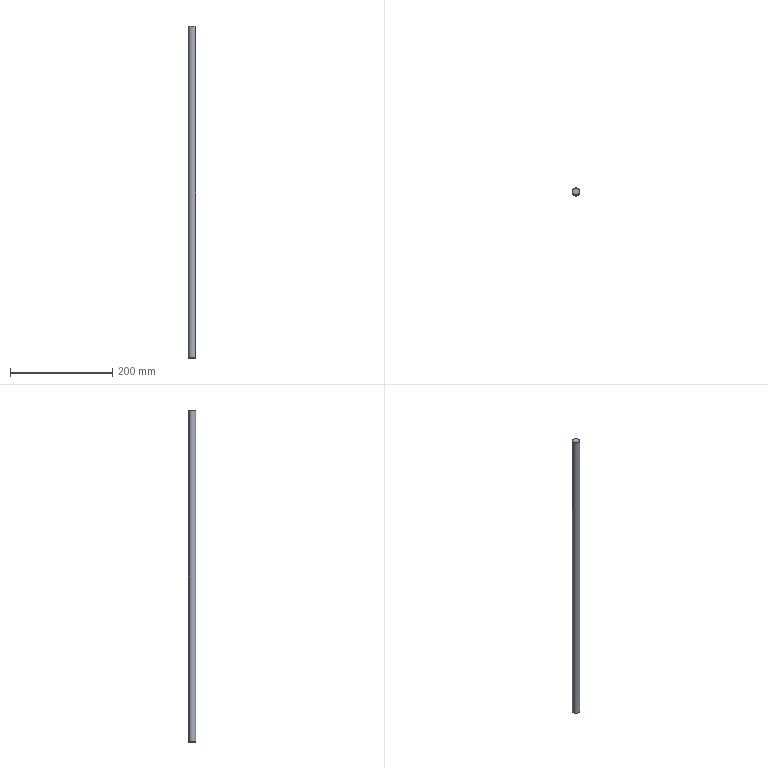Component | SolidWorks | KSD171005A-01-01-18-1 | 1 solid | 8 faces | box 15 x 15 x 650 mm | volume 114819 mm3 | cone 4 | cylinder 2 | plane 2 | commonest cylinder face diameters 15 x2
build123d program:
from build123d import *

# Parameters (mm, degrees)
SKETCH1_R           = 7.5
BOSS_EXTRUDE1_DEPTH = 650
CHAMFER1_SIZE       = 1


with BuildPart() as part:
    # Sketch1 → Boss-Extrude1 (new body)
    with BuildSketch(Plane.XY):
        Circle(SKETCH1_R)
    extrude(amount=BOSS_EXTRUDE1_DEPTH)

    # Chamfer1
    chamfer1_edges = [part.edges().sort_by_distance(p)[0] for p in [
        (-7.5, 0, 0),
        (-7.5, 0, 650),
    ]]
    chamfer(chamfer1_edges, length=CHAMFER1_SIZE)


solid = part.part

# Placed as in the assembly
solid = solid.moved(Location((-7.111, 15.73, 328), (0, 0, 0)))
STEP:
#1=COLOUR_RGB('',0.7922,0.8196,0.9333);
#2=FILL_AREA_STYLE_COLOUR('',#1);
#3=FILL_AREA_STYLE('',(#2));
#4=SURFACE_STYLE_FILL_AREA(#3);
#5=SURFACE_SIDE_STYLE('',(#4));
#6=SURFACE_STYLE_USAGE(.BOTH.,#5);
#7=PRESENTATION_STYLE_ASSIGNMENT((#6));
#8=CARTESIAN_POINT('',(-0.0646,0.4811,38.504));
#9=VERTEX_POINT('',#8);
#10=CARTESIAN_POINT('',(-0.4953,0.7575,38.504));
#11=VERTEX_POINT('',#10);
#12=CARTESIAN_POINT('',(-0.28,0.6193,38.504));
#13=DIRECTION('',(0.,0.,1.));
#14=DIRECTION('',(0.8416,-0.5401,0.));
#15=AXIS2_PLACEMENT_3D('',#12,#13,#14);
#16=CIRCLE('',#15,0.2559);
#17=EDGE_CURVE('',#9,#11,#16,.T.);
#18=ORIENTED_EDGE('',*,*,#17,.F.);
#19=CARTESIAN_POINT('',(-0.03147,0.4598,38.465));
#20=VERTEX_POINT('',#19);
#21=CARTESIAN_POINT('',(-0.0646,0.4811,38.504));
#22=DIRECTION('',(0.5951,-0.3819,-0.7071));
#23=VECTOR('',#22,39.37);
#24=LINE('',#21,#23);
#25=EDGE_CURVE('',#9,#20,#24,.T.);
#26=ORIENTED_EDGE('',*,*,#25,.T.);
#27=CARTESIAN_POINT('',(-0.5285,0.7788,38.465));
#28=VERTEX_POINT('',#27);
#29=CARTESIAN_POINT('',(-0.28,0.6193,38.465));
#30=DIRECTION('',(0.,0.,-1.));
#31=DIRECTION('',(0.8416,-0.5401,0.));
#32=AXIS2_PLACEMENT_3D('',#29,#30,#31);
#33=CIRCLE('',#32,0.2953);
#34=EDGE_CURVE('',#28,#20,#33,.T.);
#35=ORIENTED_EDGE('',*,*,#34,.F.);
#36=CARTESIAN_POINT('',(-0.4953,0.7575,38.504));
#37=DIRECTION('',(-0.5951,0.3819,-0.7071));
#38=VECTOR('',#37,39.37);
#39=LINE('',#36,#38);
#40=EDGE_CURVE('',#11,#28,#39,.T.);
#41=ORIENTED_EDGE('',*,*,#40,.F.);
#42=EDGE_LOOP('',(#18,#26,#35,#41));
#43=FACE_OUTER_BOUND('',#42,.T.);
#44=CARTESIAN_POINT('',(-0.28,0.6193,38.504));
#45=DIRECTION('',(0.,0.,-1.));
#46=DIRECTION('',(-0.8416,0.5401,0.));
#47=AXIS2_PLACEMENT_3D('',#44,#45,#46);
#48=CONICAL_SURFACE('',#47,0.2559,0.7854);
#49=ADVANCED_FACE('',(#43),#48,.T.);
#50=CARTESIAN_POINT('',(-0.4953,0.7575,12.913));
#51=VERTEX_POINT('',#50);
#52=CARTESIAN_POINT('',(-0.0646,0.4811,12.913));
#53=VERTEX_POINT('',#52);
#54=CARTESIAN_POINT('',(-0.28,0.6193,12.913));
#55=DIRECTION('',(0.,0.,-1.));
#56=DIRECTION('',(0.8416,-0.5401,0.));
#57=AXIS2_PLACEMENT_3D('',#54,#55,#56);
#58=CIRCLE('',#57,0.2559);
#59=EDGE_CURVE('',#51,#53,#58,.T.);
#60=ORIENTED_EDGE('',*,*,#59,.F.);
#61=CARTESIAN_POINT('',(-0.5285,0.7788,12.953));
#62=VERTEX_POINT('',#61);
#63=CARTESIAN_POINT('',(-0.5285,0.7788,12.953));
#64=DIRECTION('',(-0.5951,0.3819,0.7071));
#65=VECTOR('',#64,39.37);
#66=LINE('',#63,#65);
#67=EDGE_CURVE('',#51,#62,#66,.T.);
#68=ORIENTED_EDGE('',*,*,#67,.T.);
#69=CARTESIAN_POINT('',(-0.03147,0.4598,12.953));
#70=VERTEX_POINT('',#69);
#71=CARTESIAN_POINT('',(-0.28,0.6193,12.953));
#72=DIRECTION('',(0.,0.,1.));
#73=DIRECTION('',(0.8416,-0.5401,0.));
#74=AXIS2_PLACEMENT_3D('',#71,#72,#73);
#75=CIRCLE('',#74,0.2953);
#76=EDGE_CURVE('',#70,#62,#75,.T.);
#77=ORIENTED_EDGE('',*,*,#76,.F.);
#78=CARTESIAN_POINT('',(-0.03147,0.4598,12.953));
#79=DIRECTION('',(0.5951,-0.3819,0.7071));
#80=VECTOR('',#79,39.37);
#81=LINE('',#78,#80);
#82=EDGE_CURVE('',#53,#70,#81,.T.);
#83=ORIENTED_EDGE('',*,*,#82,.F.);
#84=EDGE_LOOP('',(#60,#68,#77,#83));
#85=FACE_OUTER_BOUND('',#84,.T.);
#86=CARTESIAN_POINT('',(-0.28,0.6193,12.953));
#87=DIRECTION('',(0.,0.,1.));
#88=DIRECTION('',(0.8416,-0.5401,0.));
#89=AXIS2_PLACEMENT_3D('',#86,#87,#88);
#90=CONICAL_SURFACE('',#89,0.2953,0.7854);
#91=ADVANCED_FACE('',(#85),#90,.T.);
#92=ORIENTED_EDGE('',*,*,#34,.T.);
#93=CARTESIAN_POINT('',(-0.03147,0.4598,38.504));
#94=DIRECTION('',(0.,0.,-1.));
#95=VECTOR('',#94,39.37);
#96=LINE('',#93,#95);
#97=EDGE_CURVE('',#20,#70,#96,.T.);
#98=ORIENTED_EDGE('',*,*,#97,.T.);
#99=ORIENTED_EDGE('',*,*,#76,.T.);
#100=CARTESIAN_POINT('',(-0.5285,0.7788,38.504));
#101=DIRECTION('',(0.,0.,-1.));
#102=VECTOR('',#101,39.37);
#103=LINE('',#100,#102);
#104=EDGE_CURVE('',#28,#62,#103,.T.);
#105=ORIENTED_EDGE('',*,*,#104,.F.);
#106=EDGE_LOOP('',(#92,#98,#99,#105));
#107=FACE_OUTER_BOUND('',#106,.T.);
#108=CARTESIAN_POINT('',(-0.28,0.6193,38.504));
#109=DIRECTION('',(0.,0.,-1.));
#110=DIRECTION('',(-0.8416,0.5401,0.));
#111=AXIS2_PLACEMENT_3D('',#108,#109,#110);
#112=CYLINDRICAL_SURFACE('',#111,0.2953);
#113=ADVANCED_FACE('',(#107),#112,.T.);
#114=ORIENTED_EDGE('',*,*,#97,.F.);
#115=CARTESIAN_POINT('',(-0.28,0.6193,38.465));
#116=DIRECTION('',(0.,0.,-1.));
#117=DIRECTION('',(0.8416,-0.5401,0.));
#118=AXIS2_PLACEMENT_3D('',#115,#116,#117);
#119=CIRCLE('',#118,0.2953);
#120=EDGE_CURVE('',#20,#28,#119,.T.);
#121=ORIENTED_EDGE('',*,*,#120,.T.);
#122=ORIENTED_EDGE('',*,*,#104,.T.);
#123=CARTESIAN_POINT('',(-0.28,0.6193,12.953));
#124=DIRECTION('',(0.,0.,1.));
#125=DIRECTION('',(0.8416,-0.5401,0.));
#126=AXIS2_PLACEMENT_3D('',#123,#124,#125);
#127=CIRCLE('',#126,0.2953);
#128=EDGE_CURVE('',#62,#70,#127,.T.);
#129=ORIENTED_EDGE('',*,*,#128,.T.);
#130=EDGE_LOOP('',(#114,#121,#122,#129));
#131=FACE_OUTER_BOUND('',#130,.T.);
#132=CARTESIAN_POINT('',(-0.28,0.6193,38.504));
#133=DIRECTION('',(0.,0.,-1.));
#134=DIRECTION('',(-0.8416,0.5401,0.));
#135=AXIS2_PLACEMENT_3D('',#132,#133,#134);
#136=CYLINDRICAL_SURFACE('',#135,0.2953);
#137=ADVANCED_FACE('',(#131),#136,.T.);
#138=CARTESIAN_POINT('',(-0.28,0.6193,38.504));
#139=DIRECTION('',(0.,0.,1.));
#140=DIRECTION('',(0.8416,-0.5401,0.));
#141=AXIS2_PLACEMENT_3D('',#138,#139,#140);
#142=CIRCLE('',#141,0.2559);
#143=EDGE_CURVE('',#11,#9,#142,.T.);
#144=ORIENTED_EDGE('',*,*,#143,.T.);
#145=ORIENTED_EDGE('',*,*,#17,.T.);
#146=EDGE_LOOP('',(#144,#145));
#147=FACE_OUTER_BOUND('',#146,.T.);
#148=CARTESIAN_POINT('',(-0.28,0.6193,38.504));
#149=DIRECTION('',(0.,0.,1.));
#150=DIRECTION('',(0.8416,-0.5401,0.));
#151=AXIS2_PLACEMENT_3D('',#148,#149,#150);
#152=PLANE('',#151);
#153=ADVANCED_FACE('',(#147),#152,.T.);
#154=CARTESIAN_POINT('',(-0.28,0.6193,12.913));
#155=DIRECTION('',(0.,0.,-1.));
#156=DIRECTION('',(0.8416,-0.5401,0.));
#157=AXIS2_PLACEMENT_3D('',#154,#155,#156);
#158=CIRCLE('',#157,0.2559);
#159=EDGE_CURVE('',#53,#51,#158,.T.);
#160=ORIENTED_EDGE('',*,*,#159,.T.);
#161=ORIENTED_EDGE('',*,*,#59,.T.);
#162=EDGE_LOOP('',(#160,#161));
#163=FACE_OUTER_BOUND('',#162,.T.);
#164=CARTESIAN_POINT('',(-0.28,0.6193,12.913));
#165=DIRECTION('',(0.,0.,1.));
#166=DIRECTION('',(0.8416,-0.5401,0.));
#167=AXIS2_PLACEMENT_3D('',#164,#165,#166);
#168=PLANE('',#167);
#169=ADVANCED_FACE('',(#163),#168,.F.);
#170=ORIENTED_EDGE('',*,*,#67,.F.);
#171=ORIENTED_EDGE('',*,*,#159,.F.);
#172=ORIENTED_EDGE('',*,*,#82,.T.);
#173=ORIENTED_EDGE('',*,*,#128,.F.);
#174=EDGE_LOOP('',(#170,#171,#172,#173));
#175=FACE_OUTER_BOUND('',#174,.T.);
#176=CARTESIAN_POINT('',(-0.28,0.6193,12.953));
#177=DIRECTION('',(0.,0.,1.));
#178=DIRECTION('',(0.8416,-0.5401,0.));
#179=AXIS2_PLACEMENT_3D('',#176,#177,#178);
#180=CONICAL_SURFACE('',#179,0.2953,0.7854);
#181=ADVANCED_FACE('',(#175),#180,.T.);
#182=ORIENTED_EDGE('',*,*,#25,.F.);
#183=ORIENTED_EDGE('',*,*,#143,.F.);
#184=ORIENTED_EDGE('',*,*,#40,.T.);
#185=ORIENTED_EDGE('',*,*,#120,.F.);
#186=EDGE_LOOP('',(#182,#183,#184,#185));
#187=FACE_OUTER_BOUND('',#186,.T.);
#188=CARTESIAN_POINT('',(-0.28,0.6193,38.504));
#189=DIRECTION('',(0.,0.,-1.));
#190=DIRECTION('',(-0.8416,0.5401,0.));
#191=AXIS2_PLACEMENT_3D('',#188,#189,#190);
#192=CONICAL_SURFACE('',#191,0.2559,0.7854);
#193=ADVANCED_FACE('',(#187),#192,.T.);
#194=CLOSED_SHELL('',(#49,#91,#113,#137,#153,#169,#181,#193));
#195=MANIFOLD_SOLID_BREP('',#194);
#196=STYLED_ITEM('',(#7),#195);
#197=PRESENTATION_LAYER_ASSIGNMENT('','',(#196));
#198=(LENGTH_UNIT()NAMED_UNIT(*)SI_UNIT($,.METRE.));
#199=LENGTH_MEASURE_WITH_UNIT(LENGTH_MEASURE(0.0254),#198);
#200=DIMENSIONAL_EXPONENTS(1.,0.,0.,0.,0.,0.,0.);
#201=(CONVERSION_BASED_UNIT('',#199)LENGTH_UNIT()NAMED_UNIT(#200));
#202=UNCERTAINTY_MEASURE_WITH_UNIT(LENGTH_MEASURE(0.00001),#201,'','');
#203=(NAMED_UNIT(*)PLANE_ANGLE_UNIT()SI_UNIT($,.RADIAN.));
#204=(NAMED_UNIT(*)SI_UNIT($,.STERADIAN.)SOLID_ANGLE_UNIT());
#205=(GEOMETRIC_REPRESENTATION_CONTEXT(3)GLOBAL_UNCERTAINTY_ASSIGNED_CONTEXT((#202))GLOBAL_UNIT_ASSIGNED_CONTEXT((#201,#203,#204))REPRESENTATION_CONTEXT('',''));
#206=MECHANICAL_DESIGN_GEOMETRIC_PRESENTATION_REPRESENTATION('',(#196),#205);
#207=CARTESIAN_POINT('',(0.,0.,0.));
#208=DIRECTION('',(0.,0.,1.));
#209=DIRECTION('',(1.,0.,0.));
#210=AXIS2_PLACEMENT_3D('',#207,#208,#209);
#211=(LENGTH_UNIT()NAMED_UNIT(*)SI_UNIT($,.METRE.));
#212=LENGTH_MEASURE_WITH_UNIT(LENGTH_MEASURE(0.0254),#211);
#213=DIMENSIONAL_EXPONENTS(1.,0.,0.,0.,0.,0.,0.);
#214=(CONVERSION_BASED_UNIT('',#212)LENGTH_UNIT()NAMED_UNIT(#213));
#215=UNCERTAINTY_MEASURE_WITH_UNIT(LENGTH_MEASURE(0.00001),#214,'','');
#216=(NAMED_UNIT(*)PLANE_ANGLE_UNIT()SI_UNIT($,.RADIAN.));
#217=(NAMED_UNIT(*)SI_UNIT($,.STERADIAN.)SOLID_ANGLE_UNIT());
#218=(GEOMETRIC_REPRESENTATION_CONTEXT(3)GLOBAL_UNCERTAINTY_ASSIGNED_CONTEXT((#215))GLOBAL_UNIT_ASSIGNED_CONTEXT((#214,#216,#217))REPRESENTATION_CONTEXT('',''));
#219=ADVANCED_BREP_SHAPE_REPRESENTATION('',(#195,#210),#218);